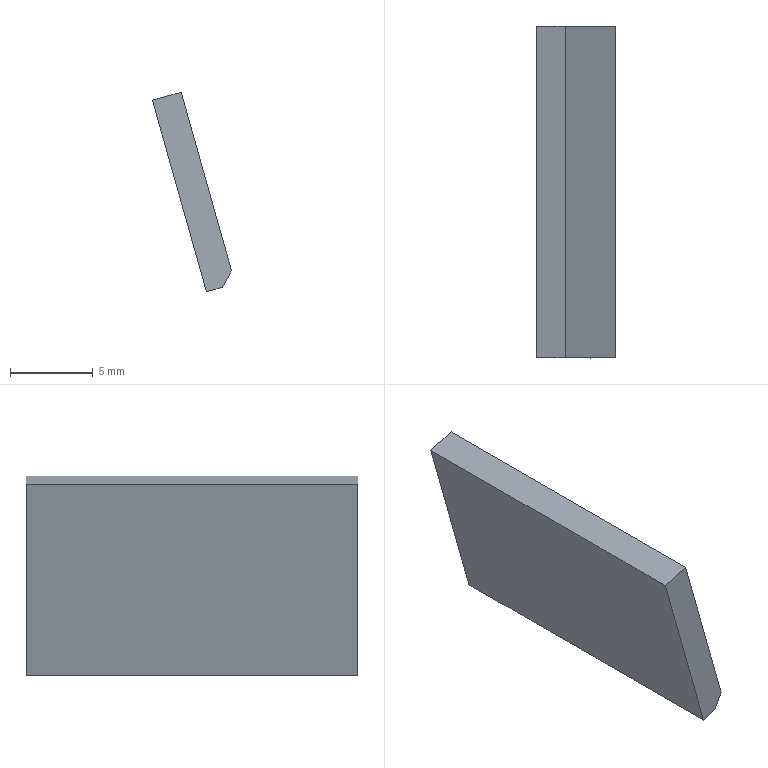Component | SolidWorks | 3-1 | 1 solid | 7 faces | box 4.77 x 20 x 12.04 mm | volume 426 mm3 | plane 7
build123d program:
from build123d import *

# Parameters (mm, degrees)
SKETCH1_W           = 12
SKETCH1_H           = 20
BOSS_EXTRUDE1_DEPTH = 1.8
CUT_EXTRUDE1_DEPTH  = 26.8


with BuildPart() as part:
    # Sketch1 → Boss-Extrude1 (new body)
    with BuildSketch(Plane(origin=(0, 0, 0), x_dir=(1, 0, 0), z_dir=(0, 1, 0))):
        Rectangle(SKETCH1_W, SKETCH1_H)
    extrude(amount=BOSS_EXTRUDE1_DEPTH)

    # Sketch2 → Cut-Extrude1 (cut)
    with BuildSketch(Plane.XY.offset(10)):
        Polygon((-5.2, 1.8), (-6, 1), (-6, 1.8), align=None)
    extrude(amount=-CUT_EXTRUDE1_DEPTH, mode=Mode.SUBTRACT)


solid = part.part

# Placed as in the assembly
solid = solid.moved(Location((1.715, 30.52, -23.113), (-90, 0, -105.722)))
STEP:
#1=CARTESIAN_POINT('',(0.003521,1.595,-0.6826));
#2=VERTEX_POINT('',#1);
#3=CARTESIAN_POINT('',(0.003521,0.8079,-0.6826));
#4=VERTEX_POINT('',#3);
#5=CARTESIAN_POINT('',(0.003521,1.595,-0.6826));
#6=DIRECTION('',(0.,-1.,-0.));
#7=VECTOR('',#6,39.37);
#8=LINE('',#5,#7);
#9=EDGE_CURVE('',#2,#4,#8,.T.);
#10=ORIENTED_EDGE('',*,*,#9,.T.);
#11=CARTESIAN_POINT('',(0.07174,0.8079,-0.6634));
#12=VERTEX_POINT('',#11);
#13=CARTESIAN_POINT('',(0.07174,0.8079,-0.6634));
#14=DIRECTION('',(-0.9626,-0.,-0.271));
#15=VECTOR('',#14,39.37);
#16=LINE('',#13,#15);
#17=EDGE_CURVE('',#12,#4,#16,.T.);
#18=ORIENTED_EDGE('',*,*,#17,.F.);
#19=CARTESIAN_POINT('',(0.07174,1.595,-0.6634));
#20=VERTEX_POINT('',#19);
#21=CARTESIAN_POINT('',(0.07174,1.595,-0.6634));
#22=DIRECTION('',(0.,-1.,-0.));
#23=VECTOR('',#22,39.37);
#24=LINE('',#21,#23);
#25=EDGE_CURVE('',#20,#12,#24,.T.);
#26=ORIENTED_EDGE('',*,*,#25,.F.);
#27=CARTESIAN_POINT('',(0.07174,1.595,-0.6634));
#28=DIRECTION('',(-0.9626,-0.,-0.271));
#29=VECTOR('',#28,39.37);
#30=LINE('',#27,#29);
#31=EDGE_CURVE('',#20,#2,#30,.T.);
#32=ORIENTED_EDGE('',*,*,#31,.T.);
#33=EDGE_LOOP('',(#10,#18,#26,#32));
#34=FACE_OUTER_BOUND('',#33,.T.);
#35=CARTESIAN_POINT('',(0.07174,1.595,-0.6634));
#36=DIRECTION('',(0.271,0.,-0.9626));
#37=DIRECTION('',(-0.,1.,0.));
#38=AXIS2_PLACEMENT_3D('',#35,#36,#37);
#39=PLANE('',#38);
#40=ADVANCED_FACE('',(#34),#39,.F.);
#41=CARTESIAN_POINT('',(0.1694,0.8079,-1.127));
#42=VERTEX_POINT('',#41);
#43=CARTESIAN_POINT('',(0.1315,0.8079,-1.137));
#44=VERTEX_POINT('',#43);
#45=CARTESIAN_POINT('',(0.1998,0.8079,-1.118));
#46=DIRECTION('',(-0.9626,-0.,-0.271));
#47=VECTOR('',#46,39.37);
#48=LINE('',#45,#47);
#49=EDGE_CURVE('',#42,#44,#48,.T.);
#50=ORIENTED_EDGE('',*,*,#49,.F.);
#51=CARTESIAN_POINT('',(0.1912,0.8079,-1.088));
#52=VERTEX_POINT('',#51);
#53=CARTESIAN_POINT('',(0.1803,0.8079,-1.107));
#54=DIRECTION('',(0.4891,-0.,0.8723));
#55=VECTOR('',#54,39.37);
#56=LINE('',#53,#55);
#57=EDGE_CURVE('',#42,#52,#56,.T.);
#58=ORIENTED_EDGE('',*,*,#57,.T.);
#59=CARTESIAN_POINT('',(0.1998,0.8079,-1.118));
#60=DIRECTION('',(0.271,0.,-0.9626));
#61=VECTOR('',#60,39.37);
#62=LINE('',#59,#61);
#63=EDGE_CURVE('',#12,#52,#62,.T.);
#64=ORIENTED_EDGE('',*,*,#63,.F.);
#65=ORIENTED_EDGE('',*,*,#17,.T.);
#66=CARTESIAN_POINT('',(0.1315,0.8079,-1.137));
#67=DIRECTION('',(0.271,0.,-0.9626));
#68=VECTOR('',#67,39.37);
#69=LINE('',#66,#68);
#70=EDGE_CURVE('',#4,#44,#69,.T.);
#71=ORIENTED_EDGE('',*,*,#70,.T.);
#72=EDGE_LOOP('',(#50,#58,#64,#65,#71));
#73=FACE_OUTER_BOUND('',#72,.T.);
#74=CARTESIAN_POINT('',(0.1998,0.8079,-1.118));
#75=DIRECTION('',(-0.,1.,0.));
#76=DIRECTION('',(-0.271,-0.,0.9626));
#77=AXIS2_PLACEMENT_3D('',#74,#75,#76);
#78=PLANE('',#77);
#79=ADVANCED_FACE('',(#73),#78,.F.);
#80=CARTESIAN_POINT('',(0.1694,1.595,-1.127));
#81=VERTEX_POINT('',#80);
#82=CARTESIAN_POINT('',(0.1315,1.595,-1.137));
#83=VERTEX_POINT('',#82);
#84=CARTESIAN_POINT('',(0.1998,1.595,-1.118));
#85=DIRECTION('',(-0.9626,-0.,-0.271));
#86=VECTOR('',#85,39.37);
#87=LINE('',#84,#86);
#88=EDGE_CURVE('',#81,#83,#87,.T.);
#89=ORIENTED_EDGE('',*,*,#88,.F.);
#90=CARTESIAN_POINT('',(0.1694,0.5401,-1.127));
#91=DIRECTION('',(-0.,1.,0.));
#92=VECTOR('',#91,39.37);
#93=LINE('',#90,#92);
#94=EDGE_CURVE('',#42,#81,#93,.T.);
#95=ORIENTED_EDGE('',*,*,#94,.F.);
#96=ORIENTED_EDGE('',*,*,#49,.T.);
#97=CARTESIAN_POINT('',(0.1315,1.595,-1.137));
#98=DIRECTION('',(-0.,1.,0.));
#99=VECTOR('',#98,39.37);
#100=LINE('',#97,#99);
#101=EDGE_CURVE('',#44,#83,#100,.T.);
#102=ORIENTED_EDGE('',*,*,#101,.T.);
#103=EDGE_LOOP('',(#89,#95,#96,#102));
#104=FACE_OUTER_BOUND('',#103,.T.);
#105=CARTESIAN_POINT('',(0.1998,1.595,-1.118));
#106=DIRECTION('',(-0.271,-0.,0.9626));
#107=DIRECTION('',(0.,-1.,-0.));
#108=AXIS2_PLACEMENT_3D('',#105,#106,#107);
#109=PLANE('',#108);
#110=ADVANCED_FACE('',(#104),#109,.F.);
#111=CARTESIAN_POINT('',(0.1912,1.595,-1.088));
#112=VERTEX_POINT('',#111);
#113=CARTESIAN_POINT('',(0.1998,1.595,-1.118));
#114=DIRECTION('',(-0.271,-0.,0.9626));
#115=VECTOR('',#114,39.37);
#116=LINE('',#113,#115);
#117=EDGE_CURVE('',#112,#20,#116,.T.);
#118=ORIENTED_EDGE('',*,*,#117,.F.);
#119=CARTESIAN_POINT('',(0.1912,1.595,-1.088));
#120=DIRECTION('',(0.4891,-0.,0.8723));
#121=VECTOR('',#120,39.37);
#122=LINE('',#119,#121);
#123=EDGE_CURVE('',#81,#112,#122,.T.);
#124=ORIENTED_EDGE('',*,*,#123,.F.);
#125=ORIENTED_EDGE('',*,*,#88,.T.);
#126=CARTESIAN_POINT('',(0.1315,1.595,-1.137));
#127=DIRECTION('',(-0.271,-0.,0.9626));
#128=VECTOR('',#127,39.37);
#129=LINE('',#126,#128);
#130=EDGE_CURVE('',#83,#2,#129,.T.);
#131=ORIENTED_EDGE('',*,*,#130,.T.);
#132=ORIENTED_EDGE('',*,*,#31,.F.);
#133=EDGE_LOOP('',(#118,#124,#125,#131,#132));
#134=FACE_OUTER_BOUND('',#133,.T.);
#135=CARTESIAN_POINT('',(0.1998,1.595,-1.118));
#136=DIRECTION('',(0.,-1.,-0.));
#137=DIRECTION('',(0.271,0.,-0.9626));
#138=AXIS2_PLACEMENT_3D('',#135,#136,#137);
#139=PLANE('',#138);
#140=ADVANCED_FACE('',(#134),#139,.F.);
#141=ORIENTED_EDGE('',*,*,#63,.T.);
#142=CARTESIAN_POINT('',(0.1912,1.202,-1.088));
#143=DIRECTION('',(-0.,1.,0.));
#144=VECTOR('',#143,39.37);
#145=LINE('',#142,#144);
#146=EDGE_CURVE('',#52,#112,#145,.T.);
#147=ORIENTED_EDGE('',*,*,#146,.T.);
#148=ORIENTED_EDGE('',*,*,#117,.T.);
#149=ORIENTED_EDGE('',*,*,#25,.T.);
#150=EDGE_LOOP('',(#141,#147,#148,#149));
#151=FACE_OUTER_BOUND('',#150,.T.);
#152=CARTESIAN_POINT('',(0.1357,1.202,-0.8907));
#153=DIRECTION('',(-0.9626,-0.,-0.271));
#154=DIRECTION('',(0.,-1.,-0.));
#155=AXIS2_PLACEMENT_3D('',#152,#153,#154);
#156=PLANE('',#155);
#157=ADVANCED_FACE('',(#151),#156,.F.);
#158=ORIENTED_EDGE('',*,*,#9,.F.);
#159=ORIENTED_EDGE('',*,*,#130,.F.);
#160=ORIENTED_EDGE('',*,*,#101,.F.);
#161=ORIENTED_EDGE('',*,*,#70,.F.);
#162=EDGE_LOOP('',(#158,#159,#160,#161));
#163=FACE_OUTER_BOUND('',#162,.T.);
#164=CARTESIAN_POINT('',(0.06753,1.202,-0.9099));
#165=DIRECTION('',(-0.9626,-0.,-0.271));
#166=DIRECTION('',(0.,-1.,-0.));
#167=AXIS2_PLACEMENT_3D('',#164,#165,#166);
#168=PLANE('',#167);
#169=ADVANCED_FACE('',(#163),#168,.T.);
#170=ORIENTED_EDGE('',*,*,#94,.T.);
#171=ORIENTED_EDGE('',*,*,#123,.T.);
#172=ORIENTED_EDGE('',*,*,#146,.F.);
#173=ORIENTED_EDGE('',*,*,#57,.F.);
#174=EDGE_LOOP('',(#170,#171,#172,#173));
#175=FACE_OUTER_BOUND('',#174,.T.);
#176=CARTESIAN_POINT('',(0.1912,0.5401,-1.088));
#177=DIRECTION('',(-0.8723,-0.,0.4891));
#178=DIRECTION('',(0.4891,-0.,0.8723));
#179=AXIS2_PLACEMENT_3D('',#176,#177,#178);
#180=PLANE('',#179);
#181=ADVANCED_FACE('',(#175),#180,.F.);
#182=CLOSED_SHELL('',(#40,#79,#110,#140,#157,#169,#181));
#183=MANIFOLD_SOLID_BREP('',#182);
#184=CARTESIAN_POINT('',(0.,0.,0.));
#185=DIRECTION('',(0.,0.,1.));
#186=DIRECTION('',(1.,0.,0.));
#187=AXIS2_PLACEMENT_3D('',#184,#185,#186);
#188=(LENGTH_UNIT()NAMED_UNIT(*)SI_UNIT($,.METRE.));
#189=LENGTH_MEASURE_WITH_UNIT(LENGTH_MEASURE(0.0254),#188);
#190=DIMENSIONAL_EXPONENTS(1.,0.,0.,0.,0.,0.,0.);
#191=(CONVERSION_BASED_UNIT('',#189)LENGTH_UNIT()NAMED_UNIT(#190));
#192=UNCERTAINTY_MEASURE_WITH_UNIT(LENGTH_MEASURE(0.00001),#191,'','');
#193=(NAMED_UNIT(*)PLANE_ANGLE_UNIT()SI_UNIT($,.RADIAN.));
#194=(NAMED_UNIT(*)SI_UNIT($,.STERADIAN.)SOLID_ANGLE_UNIT());
#195=(GEOMETRIC_REPRESENTATION_CONTEXT(3)GLOBAL_UNCERTAINTY_ASSIGNED_CONTEXT((#192))GLOBAL_UNIT_ASSIGNED_CONTEXT((#191,#193,#194))REPRESENTATION_CONTEXT('',''));
#196=ADVANCED_BREP_SHAPE_REPRESENTATION('',(#183,#187),#195);
#197=COLOUR_RGB('',0.7922,0.8196,0.9333);
#198=FILL_AREA_STYLE_COLOUR('',#197);
#199=FILL_AREA_STYLE('',(#198));
#200=SURFACE_STYLE_FILL_AREA(#199);
#201=SURFACE_SIDE_STYLE('',(#200));
#202=SURFACE_STYLE_USAGE(.BOTH.,#201);
#203=PRESENTATION_STYLE_ASSIGNMENT((#202));
#204=STYLED_ITEM('',(#203),#183);
#205=PRESENTATION_LAYER_ASSIGNMENT('','',(#204));
#206=(LENGTH_UNIT()NAMED_UNIT(*)SI_UNIT($,.METRE.));
#207=LENGTH_MEASURE_WITH_UNIT(LENGTH_MEASURE(0.0254),#206);
#208=DIMENSIONAL_EXPONENTS(1.,0.,0.,0.,0.,0.,0.);
#209=(CONVERSION_BASED_UNIT('',#207)LENGTH_UNIT()NAMED_UNIT(#208));
#210=UNCERTAINTY_MEASURE_WITH_UNIT(LENGTH_MEASURE(0.00001),#209,'','');
#211=(NAMED_UNIT(*)PLANE_ANGLE_UNIT()SI_UNIT($,.RADIAN.));
#212=(NAMED_UNIT(*)SI_UNIT($,.STERADIAN.)SOLID_ANGLE_UNIT());
#213=(GEOMETRIC_REPRESENTATION_CONTEXT(3)GLOBAL_UNCERTAINTY_ASSIGNED_CONTEXT((#210))GLOBAL_UNIT_ASSIGNED_CONTEXT((#209,#211,#212))REPRESENTATION_CONTEXT('',''));
#214=MECHANICAL_DESIGN_GEOMETRIC_PRESENTATION_REPRESENTATION('',(#204),#213);